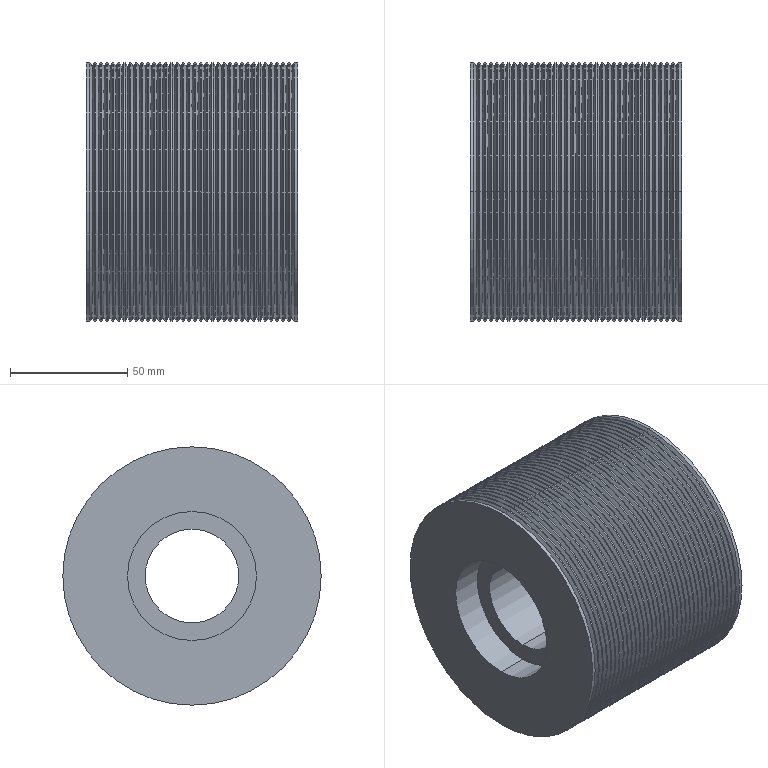Component | SolidWorks | LowerSideBeltXG-XG1-1_DrivenPulleyG.0XG-XG1-1 | 1 solid | 222 faces | box 90 x 110 x 110 mm | volume 692373 mm3 | cone 140 | cylinder 78 | plane 4 | commonest cylinder face diameters 110 x72 55 x4 40 x2
build123d program:
from build123d import *

# Parameters (mm, degrees)
LPATTERN1_COUNT = 35
LPATTERN1_PITCH = 2.5


with BuildPart() as part:
    # Sketch1 → Revolve1 (revolve)
    with BuildSketch(Plane(origin=(0, 0, 0), x_dir=(1, 0, 0), z_dir=(0, 1, 0)), mode=Mode.PRIVATE) as revolve1_sk:
        Polygon((0, 55), (90, 55), (90, 27.5), (77, 27.5), (77, 20), (13, 20), (13, 27.5), (0, 27.5), align=None)
    revolve(revolve1_sk.sketch.rotate(Axis((-694.122, 0, 0), (1, 0, 0)), 180), axis=Axis((-694.122, 0, 0), (1, 0, 0)))

    # Sketch2 → Cut-Revolve1 (revolve, cut)
    with BuildSketch(Plane(origin=(0, 0, 0), x_dir=(1, 0, 0), z_dir=(0, 1, 0)), mode=Mode.PRIVATE) as cut_revolve1_sk:
        Polygon((1.5, 55), (2.5, 53.268), (3.5, 55), align=None)
    cut_revolve1 = revolve(cut_revolve1_sk.sketch.rotate(Axis((-694.122, 0, 0), (-1, 0, 0)), 180), axis=Axis((-694.122, 0, 0), (-1, 0, 0)), mode=Mode.SUBTRACT)

    # LPattern1: Cut-Revolve1 ×35
    with Locations(*[(i * LPATTERN1_PITCH, 0, 0) for i in range(1, LPATTERN1_COUNT)]):
        add(cut_revolve1, mode=Mode.SUBTRACT)


solid = part.part

# Placed as in the assembly
solid = solid.moved(Location((-291.22, 266.5, 114), (0, 0, 0)))